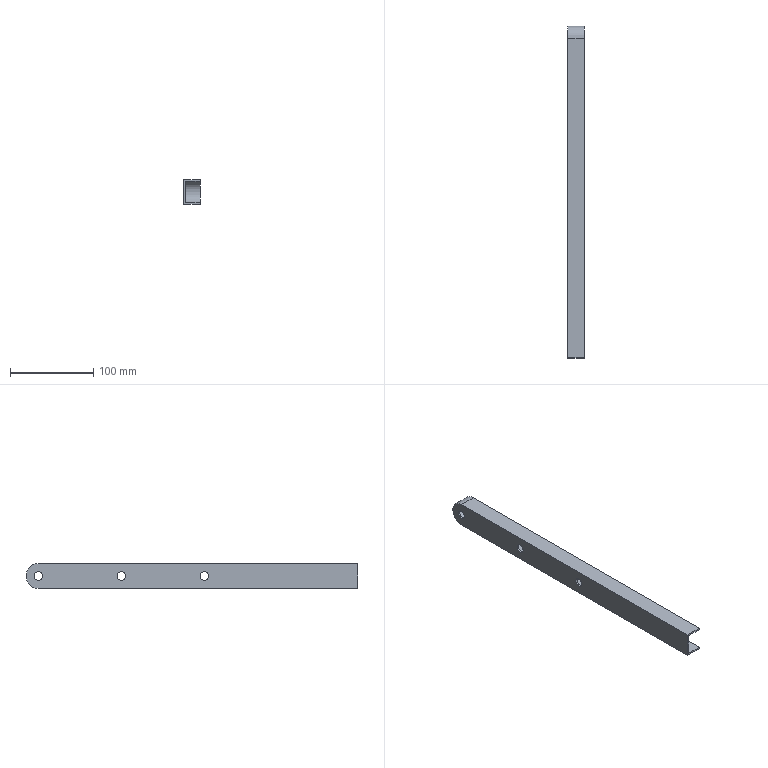Component | SolidWorks | Mirror Part4^Assembly2-2 | 1 solid | 18 faces | box 20 x 400 x 30 mm | volume 52635 mm3 | plane 10 | cylinder 8 | commonest cylinder face diameters 10 x6 30 x1 26 x1
STEP:
#1=CARTESIAN_POINT('',(-5.906,8.465,-4.74));
#2=VERTEX_POINT('',#1);
#3=CARTESIAN_POINT('',(-5.906,8.465,-4.346));
#4=VERTEX_POINT('',#3);
#5=CARTESIAN_POINT('',(-5.906,8.465,-4.543));
#6=DIRECTION('',(1.,0.,0.));
#7=DIRECTION('',(0.,0.,-1.));
#8=AXIS2_PLACEMENT_3D('',#5,#6,#7);
#9=CIRCLE('',#8,0.1969);
#10=EDGE_CURVE('',#2,#4,#9,.T.);
#11=ORIENTED_EDGE('',*,*,#10,.T.);
#12=CARTESIAN_POINT('',(-5.984,8.465,-4.346));
#13=VERTEX_POINT('',#12);
#14=CARTESIAN_POINT('',(-3.858,8.465,-4.346));
#15=DIRECTION('',(-1.,0.,0.));
#16=VECTOR('',#15,39.37);
#17=LINE('',#14,#16);
#18=EDGE_CURVE('',#4,#13,#17,.T.);
#19=ORIENTED_EDGE('',*,*,#18,.T.);
#20=CARTESIAN_POINT('',(-5.984,8.465,-4.74));
#21=VERTEX_POINT('',#20);
#22=CARTESIAN_POINT('',(-5.984,8.465,-4.543));
#23=DIRECTION('',(1.,0.,0.));
#24=DIRECTION('',(0.,0.,-1.));
#25=AXIS2_PLACEMENT_3D('',#22,#23,#24);
#26=CIRCLE('',#25,0.1969);
#27=EDGE_CURVE('',#21,#13,#26,.T.);
#28=ORIENTED_EDGE('',*,*,#27,.F.);
#29=CARTESIAN_POINT('',(-3.858,8.465,-4.74));
#30=DIRECTION('',(-1.,0.,0.));
#31=VECTOR('',#30,39.37);
#32=LINE('',#29,#31);
#33=EDGE_CURVE('',#2,#21,#32,.T.);
#34=ORIENTED_EDGE('',*,*,#33,.F.);
#35=EDGE_LOOP('',(#11,#19,#28,#34));
#36=FACE_OUTER_BOUND('',#35,.T.);
#37=CARTESIAN_POINT('',(-3.858,8.465,-4.543));
#38=DIRECTION('',(-1.,0.,0.));
#39=DIRECTION('',(0.,0.,-1.));
#40=AXIS2_PLACEMENT_3D('',#37,#38,#39);
#41=CYLINDRICAL_SURFACE('',#40,0.1969);
#42=ADVANCED_FACE('',(#36),#41,.F.);
#43=CARTESIAN_POINT('',(-5.906,12.402,-4.74));
#44=VERTEX_POINT('',#43);
#45=CARTESIAN_POINT('',(-5.906,12.402,-4.346));
#46=VERTEX_POINT('',#45);
#47=CARTESIAN_POINT('',(-5.906,12.402,-4.543));
#48=DIRECTION('',(1.,0.,0.));
#49=DIRECTION('',(0.,0.,-1.));
#50=AXIS2_PLACEMENT_3D('',#47,#48,#49);
#51=CIRCLE('',#50,0.1969);
#52=EDGE_CURVE('',#44,#46,#51,.T.);
#53=ORIENTED_EDGE('',*,*,#52,.T.);
#54=CARTESIAN_POINT('',(-5.984,12.402,-4.346));
#55=VERTEX_POINT('',#54);
#56=CARTESIAN_POINT('',(-3.858,12.402,-4.346));
#57=DIRECTION('',(-1.,0.,0.));
#58=VECTOR('',#57,39.37);
#59=LINE('',#56,#58);
#60=EDGE_CURVE('',#46,#55,#59,.T.);
#61=ORIENTED_EDGE('',*,*,#60,.T.);
#62=CARTESIAN_POINT('',(-5.984,12.402,-4.74));
#63=VERTEX_POINT('',#62);
#64=CARTESIAN_POINT('',(-5.984,12.402,-4.543));
#65=DIRECTION('',(1.,0.,0.));
#66=DIRECTION('',(0.,0.,-1.));
#67=AXIS2_PLACEMENT_3D('',#64,#65,#66);
#68=CIRCLE('',#67,0.1969);
#69=EDGE_CURVE('',#63,#55,#68,.T.);
#70=ORIENTED_EDGE('',*,*,#69,.F.);
#71=CARTESIAN_POINT('',(-3.858,12.402,-4.74));
#72=DIRECTION('',(-1.,0.,0.));
#73=VECTOR('',#72,39.37);
#74=LINE('',#71,#73);
#75=EDGE_CURVE('',#44,#63,#74,.T.);
#76=ORIENTED_EDGE('',*,*,#75,.F.);
#77=EDGE_LOOP('',(#53,#61,#70,#76));
#78=FACE_OUTER_BOUND('',#77,.T.);
#79=CARTESIAN_POINT('',(-3.858,12.402,-4.543));
#80=DIRECTION('',(-1.,0.,0.));
#81=DIRECTION('',(0.,0.,-1.));
#82=AXIS2_PLACEMENT_3D('',#79,#80,#81);
#83=CYLINDRICAL_SURFACE('',#82,0.1969);
#84=ADVANCED_FACE('',(#78),#83,.F.);
#85=CARTESIAN_POINT('',(-5.984,16.339,-4.74));
#86=VERTEX_POINT('',#85);
#87=CARTESIAN_POINT('',(-5.984,16.339,-4.346));
#88=VERTEX_POINT('',#87);
#89=CARTESIAN_POINT('',(-5.984,16.339,-4.543));
#90=DIRECTION('',(1.,0.,0.));
#91=DIRECTION('',(0.,0.,-1.));
#92=AXIS2_PLACEMENT_3D('',#89,#90,#91);
#93=CIRCLE('',#92,0.1969);
#94=EDGE_CURVE('',#86,#88,#93,.T.);
#95=ORIENTED_EDGE('',*,*,#94,.F.);
#96=CARTESIAN_POINT('',(-5.906,16.339,-4.74));
#97=VERTEX_POINT('',#96);
#98=CARTESIAN_POINT('',(-8.031,16.339,-4.74));
#99=DIRECTION('',(1.,0.,0.));
#100=VECTOR('',#99,39.37);
#101=LINE('',#98,#100);
#102=EDGE_CURVE('',#86,#97,#101,.T.);
#103=ORIENTED_EDGE('',*,*,#102,.T.);
#104=CARTESIAN_POINT('',(-5.906,16.339,-4.346));
#105=VERTEX_POINT('',#104);
#106=CARTESIAN_POINT('',(-5.906,16.339,-4.543));
#107=DIRECTION('',(-1.,0.,0.));
#108=DIRECTION('',(0.,0.,1.));
#109=AXIS2_PLACEMENT_3D('',#106,#107,#108);
#110=CIRCLE('',#109,0.1969);
#111=EDGE_CURVE('',#105,#97,#110,.T.);
#112=ORIENTED_EDGE('',*,*,#111,.F.);
#113=CARTESIAN_POINT('',(-8.031,16.339,-4.346));
#114=DIRECTION('',(1.,0.,0.));
#115=VECTOR('',#114,39.37);
#116=LINE('',#113,#115);
#117=EDGE_CURVE('',#88,#105,#116,.T.);
#118=ORIENTED_EDGE('',*,*,#117,.F.);
#119=EDGE_LOOP('',(#95,#103,#112,#118));
#120=FACE_OUTER_BOUND('',#119,.T.);
#121=CARTESIAN_POINT('',(-8.031,16.339,-4.543));
#122=DIRECTION('',(1.,0.,0.));
#123=DIRECTION('',(0.,0.,1.));
#124=AXIS2_PLACEMENT_3D('',#121,#122,#123);
#125=CYLINDRICAL_SURFACE('',#124,0.1969);
#126=ADVANCED_FACE('',(#120),#125,.F.);
#127=ORIENTED_EDGE('',*,*,#10,.F.);
#128=CARTESIAN_POINT('',(-5.906,8.465,-4.543));
#129=DIRECTION('',(1.,0.,0.));
#130=DIRECTION('',(0.,0.,-1.));
#131=AXIS2_PLACEMENT_3D('',#128,#129,#130);
#132=CIRCLE('',#131,0.1969);
#133=EDGE_CURVE('',#4,#2,#132,.T.);
#134=ORIENTED_EDGE('',*,*,#133,.F.);
#135=EDGE_LOOP('',(#127,#134));
#136=FACE_BOUND('',#135,.T.);
#137=ORIENTED_EDGE('',*,*,#52,.F.);
#138=CARTESIAN_POINT('',(-5.906,12.402,-4.543));
#139=DIRECTION('',(1.,0.,0.));
#140=DIRECTION('',(0.,0.,-1.));
#141=AXIS2_PLACEMENT_3D('',#138,#139,#140);
#142=CIRCLE('',#141,0.1969);
#143=EDGE_CURVE('',#46,#44,#142,.T.);
#144=ORIENTED_EDGE('',*,*,#143,.F.);
#145=EDGE_LOOP('',(#137,#144));
#146=FACE_BOUND('',#145,.T.);
#147=ORIENTED_EDGE('',*,*,#111,.T.);
#148=CARTESIAN_POINT('',(-5.906,16.339,-4.543));
#149=DIRECTION('',(-1.,0.,0.));
#150=DIRECTION('',(0.,0.,1.));
#151=AXIS2_PLACEMENT_3D('',#148,#149,#150);
#152=CIRCLE('',#151,0.1969);
#153=EDGE_CURVE('',#97,#105,#152,.T.);
#154=ORIENTED_EDGE('',*,*,#153,.T.);
#155=EDGE_LOOP('',(#147,#154));
#156=FACE_BOUND('',#155,.T.);
#157=CARTESIAN_POINT('',(-5.906,16.418,-5.055));
#158=VERTEX_POINT('',#157);
#159=CARTESIAN_POINT('',(-5.906,16.418,-5.049));
#160=VERTEX_POINT('',#159);
#161=CARTESIAN_POINT('',(-5.906,16.418,-5.128));
#162=DIRECTION('',(0.,0.,1.));
#163=VECTOR('',#162,39.37);
#164=LINE('',#161,#163);
#165=EDGE_CURVE('',#158,#160,#164,.T.);
#166=ORIENTED_EDGE('',*,*,#165,.T.);
#167=CARTESIAN_POINT('',(-5.906,16.418,-4.038));
#168=VERTEX_POINT('',#167);
#169=CARTESIAN_POINT('',(-5.906,16.339,-4.543));
#170=DIRECTION('',(1.,0.,0.));
#171=DIRECTION('',(0.,0.,1.));
#172=AXIS2_PLACEMENT_3D('',#169,#170,#171);
#173=CIRCLE('',#172,0.5118);
#174=EDGE_CURVE('',#160,#168,#173,.T.);
#175=ORIENTED_EDGE('',*,*,#174,.T.);
#176=CARTESIAN_POINT('',(-5.906,16.418,-4.031));
#177=VERTEX_POINT('',#176);
#178=CARTESIAN_POINT('',(-5.906,16.418,-4.038));
#179=DIRECTION('',(0.,0.,1.));
#180=VECTOR('',#179,39.37);
#181=LINE('',#178,#180);
#182=EDGE_CURVE('',#168,#177,#181,.T.);
#183=ORIENTED_EDGE('',*,*,#182,.T.);
#184=CARTESIAN_POINT('',(-5.906,1.181,-4.031));
#185=VERTEX_POINT('',#184);
#186=CARTESIAN_POINT('',(-5.906,16.929,-4.031));
#187=DIRECTION('',(0.,-1.,0.));
#188=VECTOR('',#187,39.37);
#189=LINE('',#186,#188);
#190=EDGE_CURVE('',#177,#185,#189,.T.);
#191=ORIENTED_EDGE('',*,*,#190,.T.);
#192=CARTESIAN_POINT('',(-5.906,1.181,-5.055));
#193=VERTEX_POINT('',#192);
#194=CARTESIAN_POINT('',(-5.906,1.181,-3.953));
#195=DIRECTION('',(0.,0.,1.));
#196=VECTOR('',#195,39.37);
#197=LINE('',#194,#196);
#198=EDGE_CURVE('',#193,#185,#197,.T.);
#199=ORIENTED_EDGE('',*,*,#198,.F.);
#200=CARTESIAN_POINT('',(-5.906,16.929,-5.055));
#201=DIRECTION('',(0.,-1.,0.));
#202=VECTOR('',#201,39.37);
#203=LINE('',#200,#202);
#204=EDGE_CURVE('',#158,#193,#203,.T.);
#205=ORIENTED_EDGE('',*,*,#204,.F.);
#206=EDGE_LOOP('',(#166,#175,#183,#191,#199,#205));
#207=FACE_OUTER_BOUND('',#206,.T.);
#208=CARTESIAN_POINT('',(-5.906,16.929,-3.953));
#209=DIRECTION('',(-1.,0.,0.));
#210=DIRECTION('',(0.,0.,-1.));
#211=AXIS2_PLACEMENT_3D('',#208,#209,#210);
#212=PLANE('',#211);
#213=ADVANCED_FACE('',(#136,#146,#156,#207),#212,.F.);
#214=CARTESIAN_POINT('',(-5.197,16.418,-4.031));
#215=VERTEX_POINT('',#214);
#216=CARTESIAN_POINT('',(-5.197,16.418,-4.031));
#217=DIRECTION('',(1.,0.,0.));
#218=VECTOR('',#217,39.37);
#219=LINE('',#216,#218);
#220=EDGE_CURVE('',#177,#215,#219,.T.);
#221=ORIENTED_EDGE('',*,*,#220,.T.);
#222=CARTESIAN_POINT('',(-5.197,1.181,-4.031));
#223=VERTEX_POINT('',#222);
#224=CARTESIAN_POINT('',(-5.197,16.929,-4.031));
#225=DIRECTION('',(0.,-1.,0.));
#226=VECTOR('',#225,39.37);
#227=LINE('',#224,#226);
#228=EDGE_CURVE('',#215,#223,#227,.T.);
#229=ORIENTED_EDGE('',*,*,#228,.T.);
#230=CARTESIAN_POINT('',(-5.197,1.181,-4.031));
#231=DIRECTION('',(1.,0.,0.));
#232=VECTOR('',#231,39.37);
#233=LINE('',#230,#232);
#234=EDGE_CURVE('',#185,#223,#233,.T.);
#235=ORIENTED_EDGE('',*,*,#234,.F.);
#236=ORIENTED_EDGE('',*,*,#190,.F.);
#237=EDGE_LOOP('',(#221,#229,#235,#236));
#238=FACE_OUTER_BOUND('',#237,.T.);
#239=CARTESIAN_POINT('',(-5.197,16.929,-4.031));
#240=DIRECTION('',(0.,0.,1.));
#241=DIRECTION('',(-1.,0.,0.));
#242=AXIS2_PLACEMENT_3D('',#239,#240,#241);
#243=PLANE('',#242);
#244=ADVANCED_FACE('',(#238),#243,.F.);
#245=CARTESIAN_POINT('',(-5.197,16.418,-5.055));
#246=VERTEX_POINT('',#245);
#247=CARTESIAN_POINT('',(-5.197,16.418,-5.055));
#248=DIRECTION('',(-1.,0.,0.));
#249=VECTOR('',#248,39.37);
#250=LINE('',#247,#249);
#251=EDGE_CURVE('',#246,#158,#250,.T.);
#252=ORIENTED_EDGE('',*,*,#251,.T.);
#253=ORIENTED_EDGE('',*,*,#204,.T.);
#254=CARTESIAN_POINT('',(-5.197,1.181,-5.055));
#255=VERTEX_POINT('',#254);
#256=CARTESIAN_POINT('',(-5.197,1.181,-5.055));
#257=DIRECTION('',(-1.,0.,0.));
#258=VECTOR('',#257,39.37);
#259=LINE('',#256,#258);
#260=EDGE_CURVE('',#255,#193,#259,.T.);
#261=ORIENTED_EDGE('',*,*,#260,.F.);
#262=CARTESIAN_POINT('',(-5.197,16.929,-5.055));
#263=DIRECTION('',(0.,-1.,0.));
#264=VECTOR('',#263,39.37);
#265=LINE('',#262,#264);
#266=EDGE_CURVE('',#246,#255,#265,.T.);
#267=ORIENTED_EDGE('',*,*,#266,.F.);
#268=EDGE_LOOP('',(#252,#253,#261,#267));
#269=FACE_OUTER_BOUND('',#268,.T.);
#270=CARTESIAN_POINT('',(-5.197,16.929,-5.055));
#271=DIRECTION('',(0.,0.,-1.));
#272=DIRECTION('',(1.,0.,0.));
#273=AXIS2_PLACEMENT_3D('',#270,#271,#272);
#274=PLANE('',#273);
#275=ADVANCED_FACE('',(#269),#274,.F.);
#276=CARTESIAN_POINT('',(-5.984,16.339,-3.953));
#277=VERTEX_POINT('',#276);
#278=CARTESIAN_POINT('',(-5.984,1.181,-3.953));
#279=VERTEX_POINT('',#278);
#280=CARTESIAN_POINT('',(-5.984,16.929,-3.953));
#281=DIRECTION('',(0.,-1.,0.));
#282=VECTOR('',#281,39.37);
#283=LINE('',#280,#282);
#284=EDGE_CURVE('',#277,#279,#283,.T.);
#285=ORIENTED_EDGE('',*,*,#284,.T.);
#286=CARTESIAN_POINT('',(-5.197,1.181,-3.953));
#287=VERTEX_POINT('',#286);
#288=CARTESIAN_POINT('',(-5.197,1.181,-3.953));
#289=DIRECTION('',(1.,0.,0.));
#290=VECTOR('',#289,39.37);
#291=LINE('',#288,#290);
#292=EDGE_CURVE('',#279,#287,#291,.T.);
#293=ORIENTED_EDGE('',*,*,#292,.T.);
#294=CARTESIAN_POINT('',(-5.197,16.339,-3.953));
#295=VERTEX_POINT('',#294);
#296=CARTESIAN_POINT('',(-5.197,16.929,-3.953));
#297=DIRECTION('',(0.,-1.,0.));
#298=VECTOR('',#297,39.37);
#299=LINE('',#296,#298);
#300=EDGE_CURVE('',#295,#287,#299,.T.);
#301=ORIENTED_EDGE('',*,*,#300,.F.);
#302=CARTESIAN_POINT('',(-3.858,16.339,-3.953));
#303=DIRECTION('',(-1.,0.,0.));
#304=VECTOR('',#303,39.37);
#305=LINE('',#302,#304);
#306=EDGE_CURVE('',#295,#277,#305,.T.);
#307=ORIENTED_EDGE('',*,*,#306,.T.);
#308=EDGE_LOOP('',(#285,#293,#301,#307));
#309=FACE_OUTER_BOUND('',#308,.T.);
#310=CARTESIAN_POINT('',(-5.197,16.929,-3.953));
#311=DIRECTION('',(0.,0.,1.));
#312=DIRECTION('',(-1.,0.,0.));
#313=AXIS2_PLACEMENT_3D('',#310,#311,#312);
#314=PLANE('',#313);
#315=ADVANCED_FACE('',(#309),#314,.T.);
#316=ORIENTED_EDGE('',*,*,#27,.T.);
#317=CARTESIAN_POINT('',(-5.984,8.465,-4.543));
#318=DIRECTION('',(1.,0.,0.));
#319=DIRECTION('',(0.,0.,-1.));
#320=AXIS2_PLACEMENT_3D('',#317,#318,#319);
#321=CIRCLE('',#320,0.1969);
#322=EDGE_CURVE('',#13,#21,#321,.T.);
#323=ORIENTED_EDGE('',*,*,#322,.T.);
#324=EDGE_LOOP('',(#316,#323));
#325=FACE_BOUND('',#324,.T.);
#326=ORIENTED_EDGE('',*,*,#69,.T.);
#327=CARTESIAN_POINT('',(-5.984,12.402,-4.543));
#328=DIRECTION('',(1.,0.,0.));
#329=DIRECTION('',(0.,0.,-1.));
#330=AXIS2_PLACEMENT_3D('',#327,#328,#329);
#331=CIRCLE('',#330,0.1969);
#332=EDGE_CURVE('',#55,#63,#331,.T.);
#333=ORIENTED_EDGE('',*,*,#332,.T.);
#334=EDGE_LOOP('',(#326,#333));
#335=FACE_BOUND('',#334,.T.);
#336=CARTESIAN_POINT('',(-5.984,16.339,-4.543));
#337=DIRECTION('',(1.,0.,0.));
#338=DIRECTION('',(0.,0.,-1.));
#339=AXIS2_PLACEMENT_3D('',#336,#337,#338);
#340=CIRCLE('',#339,0.1969);
#341=EDGE_CURVE('',#88,#86,#340,.T.);
#342=ORIENTED_EDGE('',*,*,#341,.T.);
#343=ORIENTED_EDGE('',*,*,#94,.T.);
#344=EDGE_LOOP('',(#342,#343));
#345=FACE_BOUND('',#344,.T.);
#346=CARTESIAN_POINT('',(-5.984,16.339,-5.134));
#347=VERTEX_POINT('',#346);
#348=CARTESIAN_POINT('',(-5.984,16.339,-4.543));
#349=DIRECTION('',(-1.,0.,0.));
#350=DIRECTION('',(0.,0.,-1.));
#351=AXIS2_PLACEMENT_3D('',#348,#349,#350);
#352=CIRCLE('',#351,0.5906);
#353=EDGE_CURVE('',#277,#347,#352,.T.);
#354=ORIENTED_EDGE('',*,*,#353,.T.);
#355=CARTESIAN_POINT('',(-5.984,1.181,-5.134));
#356=VERTEX_POINT('',#355);
#357=CARTESIAN_POINT('',(-5.984,16.929,-5.134));
#358=DIRECTION('',(0.,-1.,0.));
#359=VECTOR('',#358,39.37);
#360=LINE('',#357,#359);
#361=EDGE_CURVE('',#347,#356,#360,.T.);
#362=ORIENTED_EDGE('',*,*,#361,.T.);
#363=CARTESIAN_POINT('',(-5.984,1.181,-3.953));
#364=DIRECTION('',(0.,0.,1.));
#365=VECTOR('',#364,39.37);
#366=LINE('',#363,#365);
#367=EDGE_CURVE('',#356,#279,#366,.T.);
#368=ORIENTED_EDGE('',*,*,#367,.T.);
#369=ORIENTED_EDGE('',*,*,#284,.F.);
#370=EDGE_LOOP('',(#354,#362,#368,#369));
#371=FACE_OUTER_BOUND('',#370,.T.);
#372=CARTESIAN_POINT('',(-5.984,16.929,-3.953));
#373=DIRECTION('',(-1.,0.,0.));
#374=DIRECTION('',(0.,0.,-1.));
#375=AXIS2_PLACEMENT_3D('',#372,#373,#374);
#376=PLANE('',#375);
#377=ADVANCED_FACE('',(#325,#335,#345,#371),#376,.T.);
#378=CARTESIAN_POINT('',(-5.197,16.339,-5.134));
#379=VERTEX_POINT('',#378);
#380=CARTESIAN_POINT('',(-3.858,16.339,-5.134));
#381=DIRECTION('',(-1.,0.,0.));
#382=VECTOR('',#381,39.37);
#383=LINE('',#380,#382);
#384=EDGE_CURVE('',#379,#347,#383,.T.);
#385=ORIENTED_EDGE('',*,*,#384,.F.);
#386=CARTESIAN_POINT('',(-5.197,1.181,-5.134));
#387=VERTEX_POINT('',#386);
#388=CARTESIAN_POINT('',(-5.197,16.929,-5.134));
#389=DIRECTION('',(0.,-1.,0.));
#390=VECTOR('',#389,39.37);
#391=LINE('',#388,#390);
#392=EDGE_CURVE('',#379,#387,#391,.T.);
#393=ORIENTED_EDGE('',*,*,#392,.T.);
#394=CARTESIAN_POINT('',(-5.197,1.181,-5.134));
#395=DIRECTION('',(-1.,0.,0.));
#396=VECTOR('',#395,39.37);
#397=LINE('',#394,#396);
#398=EDGE_CURVE('',#387,#356,#397,.T.);
#399=ORIENTED_EDGE('',*,*,#398,.T.);
#400=ORIENTED_EDGE('',*,*,#361,.F.);
#401=EDGE_LOOP('',(#385,#393,#399,#400));
#402=FACE_OUTER_BOUND('',#401,.T.);
#403=CARTESIAN_POINT('',(-5.197,16.929,-5.134));
#404=DIRECTION('',(0.,0.,-1.));
#405=DIRECTION('',(1.,0.,0.));
#406=AXIS2_PLACEMENT_3D('',#403,#404,#405);
#407=PLANE('',#406);
#408=ADVANCED_FACE('',(#402),#407,.T.);
#409=CARTESIAN_POINT('',(-5.197,16.339,-4.543));
#410=DIRECTION('',(1.,0.,0.));
#411=DIRECTION('',(0.,0.,1.));
#412=AXIS2_PLACEMENT_3D('',#409,#410,#411);
#413=CIRCLE('',#412,0.5906);
#414=EDGE_CURVE('',#379,#295,#413,.T.);
#415=ORIENTED_EDGE('',*,*,#414,.T.);
#416=ORIENTED_EDGE('',*,*,#300,.T.);
#417=CARTESIAN_POINT('',(-5.197,1.181,-3.953));
#418=DIRECTION('',(0.,0.,-1.));
#419=VECTOR('',#418,39.37);
#420=LINE('',#417,#419);
#421=EDGE_CURVE('',#287,#223,#420,.T.);
#422=ORIENTED_EDGE('',*,*,#421,.T.);
#423=ORIENTED_EDGE('',*,*,#228,.F.);
#424=CARTESIAN_POINT('',(-5.197,16.418,-4.038));
#425=VERTEX_POINT('',#424);
#426=CARTESIAN_POINT('',(-5.197,16.418,-4.038));
#427=DIRECTION('',(0.,0.,1.));
#428=VECTOR('',#427,39.37);
#429=LINE('',#426,#428);
#430=EDGE_CURVE('',#425,#215,#429,.T.);
#431=ORIENTED_EDGE('',*,*,#430,.F.);
#432=CARTESIAN_POINT('',(-5.197,16.418,-5.049));
#433=VERTEX_POINT('',#432);
#434=CARTESIAN_POINT('',(-5.197,16.339,-4.543));
#435=DIRECTION('',(1.,0.,0.));
#436=DIRECTION('',(0.,0.,1.));
#437=AXIS2_PLACEMENT_3D('',#434,#435,#436);
#438=CIRCLE('',#437,0.5118);
#439=EDGE_CURVE('',#433,#425,#438,.T.);
#440=ORIENTED_EDGE('',*,*,#439,.F.);
#441=CARTESIAN_POINT('',(-5.197,16.418,-5.128));
#442=DIRECTION('',(0.,0.,1.));
#443=VECTOR('',#442,39.37);
#444=LINE('',#441,#443);
#445=EDGE_CURVE('',#246,#433,#444,.T.);
#446=ORIENTED_EDGE('',*,*,#445,.F.);
#447=ORIENTED_EDGE('',*,*,#266,.T.);
#448=CARTESIAN_POINT('',(-5.197,1.181,-5.055));
#449=DIRECTION('',(0.,0.,-1.));
#450=VECTOR('',#449,39.37);
#451=LINE('',#448,#450);
#452=EDGE_CURVE('',#255,#387,#451,.T.);
#453=ORIENTED_EDGE('',*,*,#452,.T.);
#454=ORIENTED_EDGE('',*,*,#392,.F.);
#455=EDGE_LOOP('',(#415,#416,#422,#423,#431,#440,#446,#447,#453,#454));
#456=FACE_OUTER_BOUND('',#455,.T.);
#457=CARTESIAN_POINT('',(-5.197,16.929,-5.055));
#458=DIRECTION('',(1.,0.,0.));
#459=DIRECTION('',(0.,0.,1.));
#460=AXIS2_PLACEMENT_3D('',#457,#458,#459);
#461=PLANE('',#460);
#462=ADVANCED_FACE('',(#456),#461,.T.);
#463=ORIENTED_EDGE('',*,*,#234,.T.);
#464=ORIENTED_EDGE('',*,*,#421,.F.);
#465=ORIENTED_EDGE('',*,*,#292,.F.);
#466=ORIENTED_EDGE('',*,*,#367,.F.);
#467=ORIENTED_EDGE('',*,*,#398,.F.);
#468=ORIENTED_EDGE('',*,*,#452,.F.);
#469=ORIENTED_EDGE('',*,*,#260,.T.);
#470=ORIENTED_EDGE('',*,*,#198,.T.);
#471=EDGE_LOOP('',(#463,#464,#465,#466,#467,#468,#469,#470));
#472=FACE_OUTER_BOUND('',#471,.T.);
#473=CARTESIAN_POINT('',(-5.984,1.181,-10.796));
#474=DIRECTION('',(0.,-1.,0.));
#475=DIRECTION('',(0.,0.,1.));
#476=AXIS2_PLACEMENT_3D('',#473,#474,#475);
#477=PLANE('',#476);
#478=ADVANCED_FACE('',(#472),#477,.T.);
#479=ORIENTED_EDGE('',*,*,#384,.T.);
#480=ORIENTED_EDGE('',*,*,#353,.F.);
#481=ORIENTED_EDGE('',*,*,#306,.F.);
#482=ORIENTED_EDGE('',*,*,#414,.F.);
#483=EDGE_LOOP('',(#479,#480,#481,#482));
#484=FACE_OUTER_BOUND('',#483,.T.);
#485=CARTESIAN_POINT('',(-3.858,16.339,-4.543));
#486=DIRECTION('',(-1.,0.,0.));
#487=DIRECTION('',(0.,0.,-1.));
#488=AXIS2_PLACEMENT_3D('',#485,#486,#487);
#489=CYLINDRICAL_SURFACE('',#488,0.5906);
#490=ADVANCED_FACE('',(#484),#489,.T.);
#491=ORIENTED_EDGE('',*,*,#445,.T.);
#492=CARTESIAN_POINT('',(-3.92,16.418,-5.049));
#493=DIRECTION('',(-1.,0.,0.));
#494=VECTOR('',#493,39.37);
#495=LINE('',#492,#494);
#496=EDGE_CURVE('',#433,#160,#495,.T.);
#497=ORIENTED_EDGE('',*,*,#496,.T.);
#498=ORIENTED_EDGE('',*,*,#165,.F.);
#499=ORIENTED_EDGE('',*,*,#251,.F.);
#500=EDGE_LOOP('',(#491,#497,#498,#499));
#501=FACE_OUTER_BOUND('',#500,.T.);
#502=CARTESIAN_POINT('',(-3.92,16.418,-5.128));
#503=DIRECTION('',(0.,1.,0.));
#504=DIRECTION('',(-1.,0.,0.));
#505=AXIS2_PLACEMENT_3D('',#502,#503,#504);
#506=PLANE('',#505);
#507=ADVANCED_FACE('',(#501),#506,.F.);
#508=ORIENTED_EDGE('',*,*,#182,.F.);
#509=CARTESIAN_POINT('',(-3.92,16.418,-4.038));
#510=DIRECTION('',(-1.,0.,0.));
#511=VECTOR('',#510,39.37);
#512=LINE('',#509,#511);
#513=EDGE_CURVE('',#425,#168,#512,.T.);
#514=ORIENTED_EDGE('',*,*,#513,.F.);
#515=ORIENTED_EDGE('',*,*,#430,.T.);
#516=ORIENTED_EDGE('',*,*,#220,.F.);
#517=EDGE_LOOP('',(#508,#514,#515,#516));
#518=FACE_OUTER_BOUND('',#517,.T.);
#519=CARTESIAN_POINT('',(-3.92,16.418,-4.038));
#520=DIRECTION('',(0.,1.,0.));
#521=DIRECTION('',(-1.,0.,0.));
#522=AXIS2_PLACEMENT_3D('',#519,#520,#521);
#523=PLANE('',#522);
#524=ADVANCED_FACE('',(#518),#523,.F.);
#525=ORIENTED_EDGE('',*,*,#439,.T.);
#526=ORIENTED_EDGE('',*,*,#513,.T.);
#527=ORIENTED_EDGE('',*,*,#174,.F.);
#528=ORIENTED_EDGE('',*,*,#496,.F.);
#529=EDGE_LOOP('',(#525,#526,#527,#528));
#530=FACE_OUTER_BOUND('',#529,.T.);
#531=CARTESIAN_POINT('',(-3.92,16.339,-4.543));
#532=DIRECTION('',(-1.,0.,0.));
#533=DIRECTION('',(0.,0.,-1.));
#534=AXIS2_PLACEMENT_3D('',#531,#532,#533);
#535=CYLINDRICAL_SURFACE('',#534,0.5118);
#536=ADVANCED_FACE('',(#530),#535,.F.);
#537=ORIENTED_EDGE('',*,*,#102,.F.);
#538=ORIENTED_EDGE('',*,*,#341,.F.);
#539=ORIENTED_EDGE('',*,*,#117,.T.);
#540=ORIENTED_EDGE('',*,*,#153,.F.);
#541=EDGE_LOOP('',(#537,#538,#539,#540));
#542=FACE_OUTER_BOUND('',#541,.T.);
#543=CARTESIAN_POINT('',(-8.031,16.339,-4.543));
#544=DIRECTION('',(1.,0.,0.));
#545=DIRECTION('',(0.,0.,1.));
#546=AXIS2_PLACEMENT_3D('',#543,#544,#545);
#547=CYLINDRICAL_SURFACE('',#546,0.1969);
#548=ADVANCED_FACE('',(#542),#547,.F.);
#549=ORIENTED_EDGE('',*,*,#60,.F.);
#550=ORIENTED_EDGE('',*,*,#143,.T.);
#551=ORIENTED_EDGE('',*,*,#75,.T.);
#552=ORIENTED_EDGE('',*,*,#332,.F.);
#553=EDGE_LOOP('',(#549,#550,#551,#552));
#554=FACE_OUTER_BOUND('',#553,.T.);
#555=CARTESIAN_POINT('',(-3.858,12.402,-4.543));
#556=DIRECTION('',(-1.,0.,0.));
#557=DIRECTION('',(0.,0.,-1.));
#558=AXIS2_PLACEMENT_3D('',#555,#556,#557);
#559=CYLINDRICAL_SURFACE('',#558,0.1969);
#560=ADVANCED_FACE('',(#554),#559,.F.);
#561=ORIENTED_EDGE('',*,*,#18,.F.);
#562=ORIENTED_EDGE('',*,*,#133,.T.);
#563=ORIENTED_EDGE('',*,*,#33,.T.);
#564=ORIENTED_EDGE('',*,*,#322,.F.);
#565=EDGE_LOOP('',(#561,#562,#563,#564));
#566=FACE_OUTER_BOUND('',#565,.T.);
#567=CARTESIAN_POINT('',(-3.858,8.465,-4.543));
#568=DIRECTION('',(-1.,0.,0.));
#569=DIRECTION('',(0.,0.,-1.));
#570=AXIS2_PLACEMENT_3D('',#567,#568,#569);
#571=CYLINDRICAL_SURFACE('',#570,0.1969);
#572=ADVANCED_FACE('',(#566),#571,.F.);
#573=CLOSED_SHELL('',(#42,#84,#126,#213,#244,#275,#315,#377,#408,#462,#478,#490,#507,#524,#536,#548,#560,#572));
#574=MANIFOLD_SOLID_BREP('',#573);
#575=CARTESIAN_POINT('',(0.,0.,0.));
#576=DIRECTION('',(0.,0.,1.));
#577=DIRECTION('',(1.,0.,0.));
#578=AXIS2_PLACEMENT_3D('',#575,#576,#577);
#579=(LENGTH_UNIT()NAMED_UNIT(*)SI_UNIT($,.METRE.));
#580=LENGTH_MEASURE_WITH_UNIT(LENGTH_MEASURE(0.0254),#579);
#581=DIMENSIONAL_EXPONENTS(1.,0.,0.,0.,0.,0.,0.);
#582=(CONVERSION_BASED_UNIT('',#580)LENGTH_UNIT()NAMED_UNIT(#581));
#583=UNCERTAINTY_MEASURE_WITH_UNIT(LENGTH_MEASURE(0.00001),#582,'','');
#584=(NAMED_UNIT(*)PLANE_ANGLE_UNIT()SI_UNIT($,.RADIAN.));
#585=(NAMED_UNIT(*)SI_UNIT($,.STERADIAN.)SOLID_ANGLE_UNIT());
#586=(GEOMETRIC_REPRESENTATION_CONTEXT(3)GLOBAL_UNCERTAINTY_ASSIGNED_CONTEXT((#583))GLOBAL_UNIT_ASSIGNED_CONTEXT((#582,#584,#585))REPRESENTATION_CONTEXT('',''));
#587=ADVANCED_BREP_SHAPE_REPRESENTATION('',(#574,#578),#586);
#588=COLOUR_RGB('',0.7922,0.8196,0.9333);
#589=FILL_AREA_STYLE_COLOUR('',#588);
#590=FILL_AREA_STYLE('',(#589));
#591=SURFACE_STYLE_FILL_AREA(#590);
#592=SURFACE_SIDE_STYLE('',(#591));
#593=SURFACE_STYLE_USAGE(.BOTH.,#592);
#594=PRESENTATION_STYLE_ASSIGNMENT((#593));
#595=STYLED_ITEM('',(#594),#574);
#596=PRESENTATION_LAYER_ASSIGNMENT('','',(#595));
#597=(LENGTH_UNIT()NAMED_UNIT(*)SI_UNIT($,.METRE.));
#598=LENGTH_MEASURE_WITH_UNIT(LENGTH_MEASURE(0.0254),#597);
#599=DIMENSIONAL_EXPONENTS(1.,0.,0.,0.,0.,0.,0.);
#600=(CONVERSION_BASED_UNIT('',#598)LENGTH_UNIT()NAMED_UNIT(#599));
#601=UNCERTAINTY_MEASURE_WITH_UNIT(LENGTH_MEASURE(0.00001),#600,'','');
#602=(NAMED_UNIT(*)PLANE_ANGLE_UNIT()SI_UNIT($,.RADIAN.));
#603=(NAMED_UNIT(*)SI_UNIT($,.STERADIAN.)SOLID_ANGLE_UNIT());
#604=(GEOMETRIC_REPRESENTATION_CONTEXT(3)GLOBAL_UNCERTAINTY_ASSIGNED_CONTEXT((#601))GLOBAL_UNIT_ASSIGNED_CONTEXT((#600,#602,#603))REPRESENTATION_CONTEXT('',''));
#605=MECHANICAL_DESIGN_GEOMETRIC_PRESENTATION_REPRESENTATION('',(#595),#604);